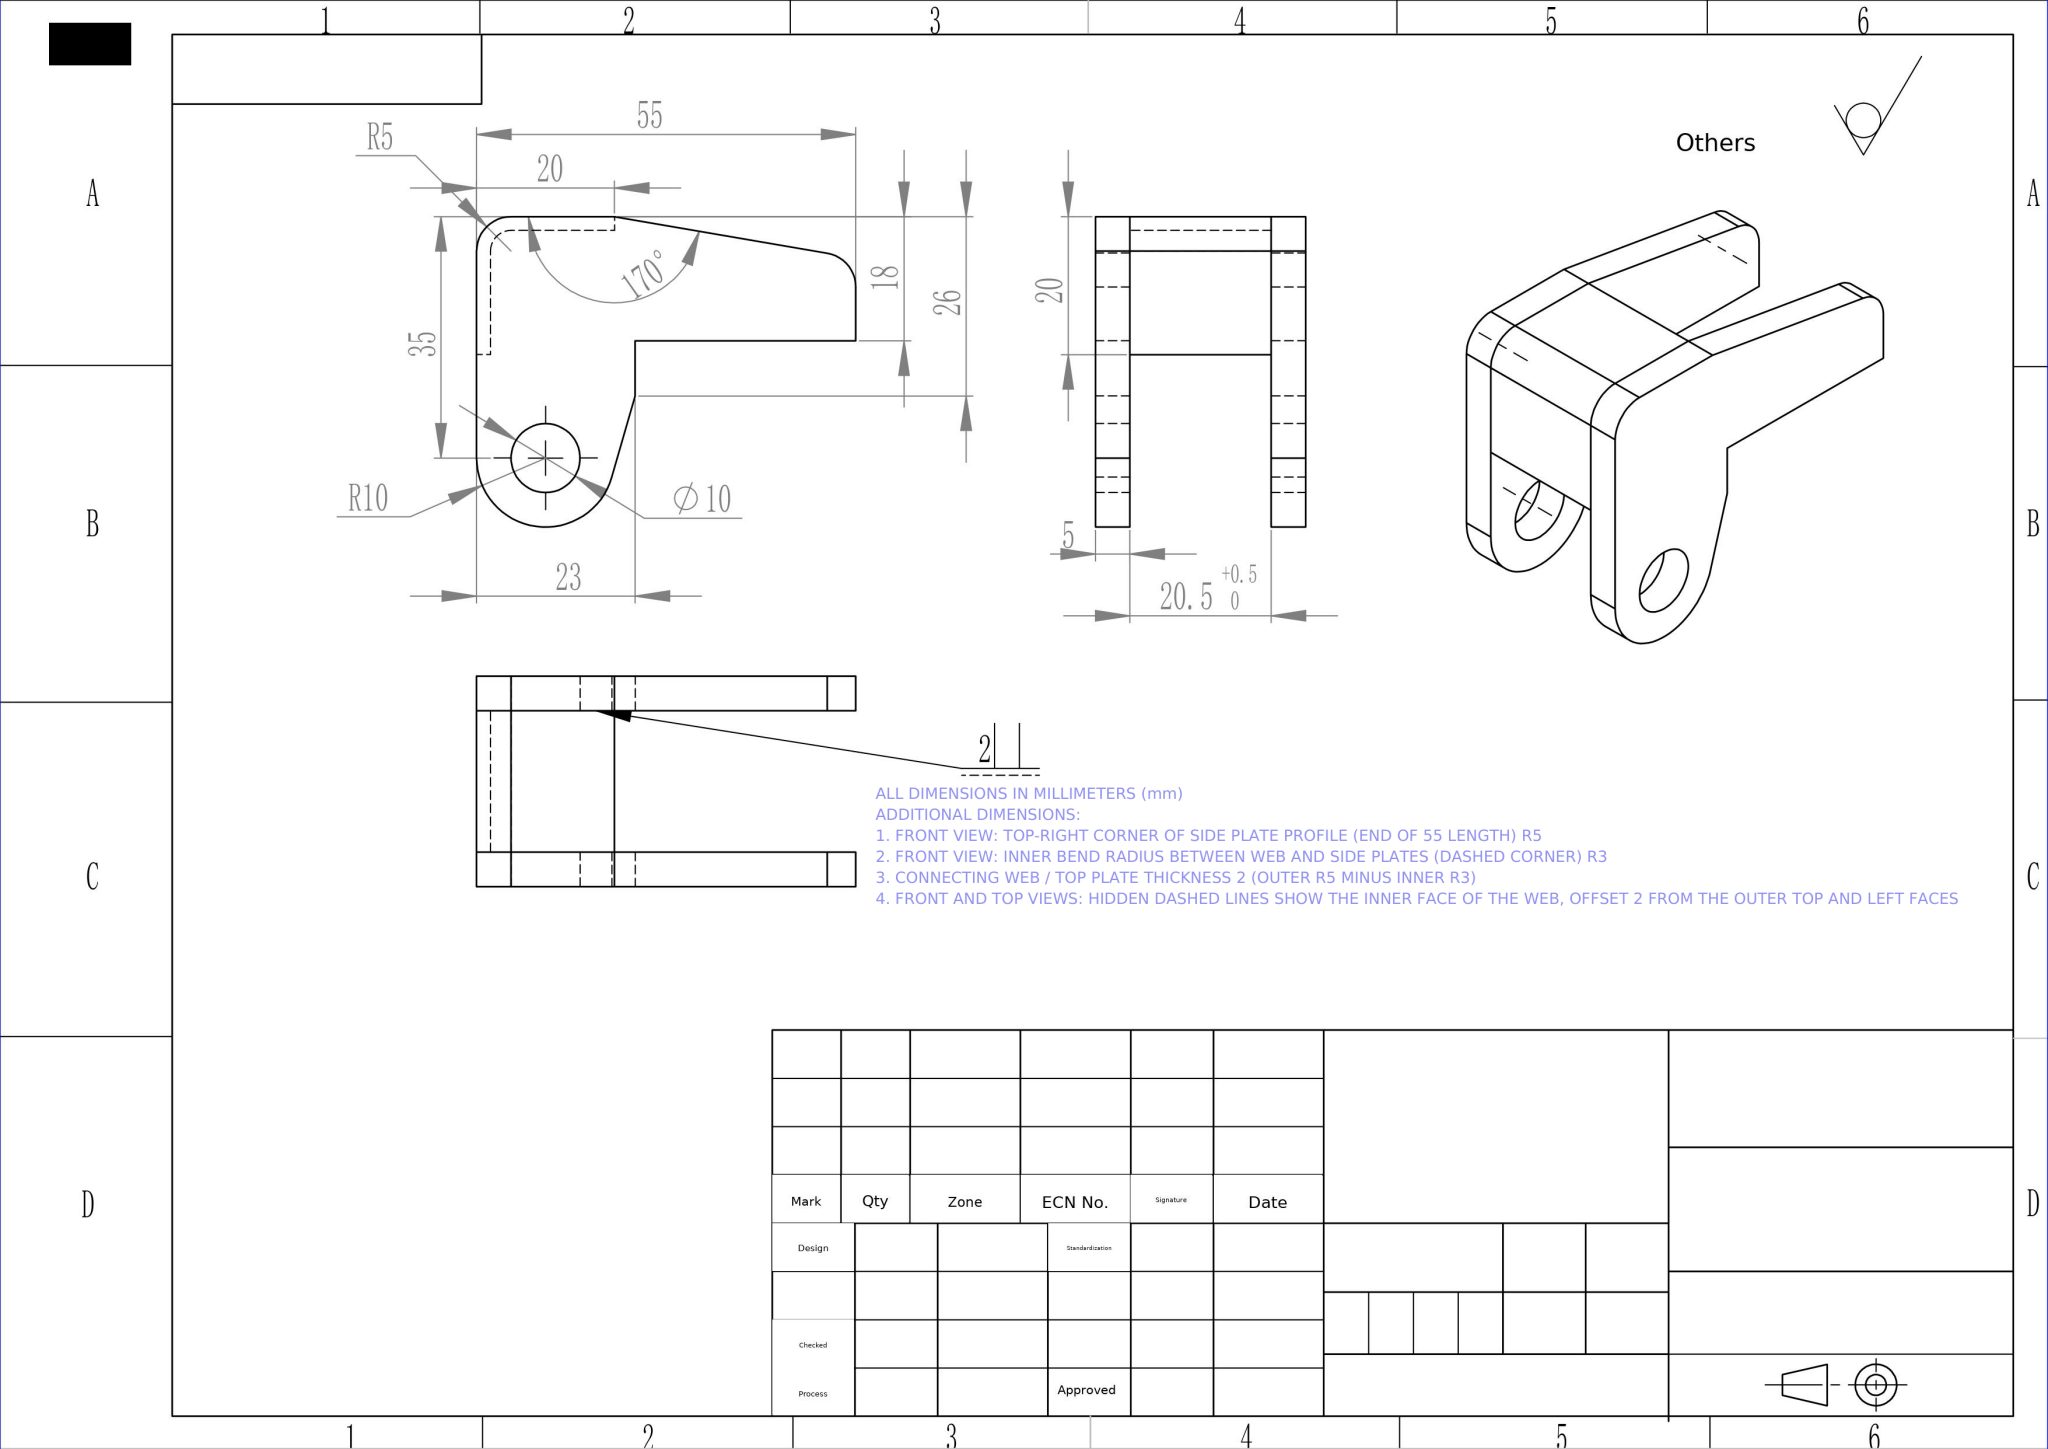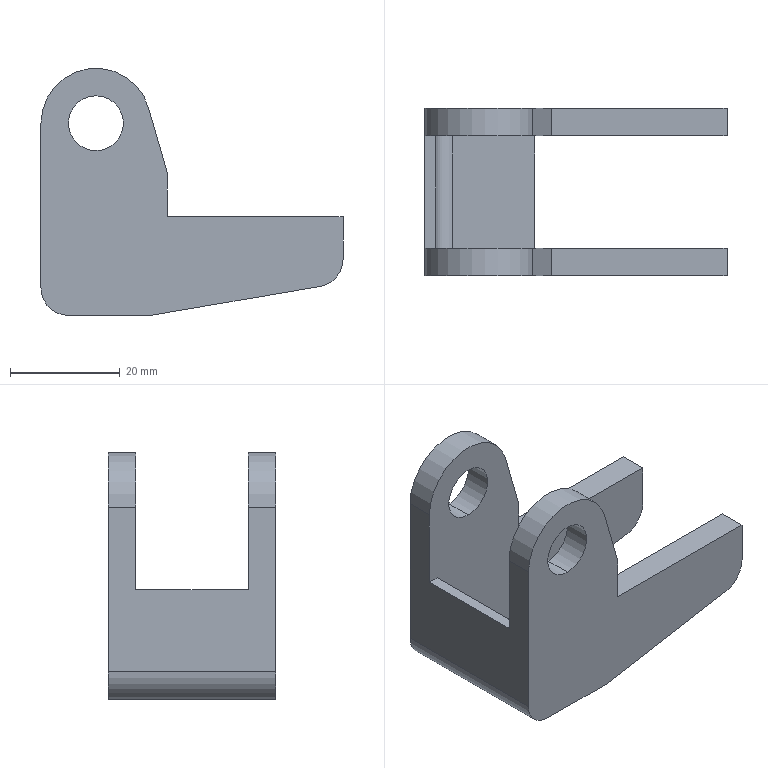Part | NX | mm | 1 solid | 30 faces | box 55 x 30.5 x 45 mm | volume 14831 mm3 | plane 20 | cylinder 10 | commonest cylinder face diameters 10 x7 20 x2 6 x1
STEP:
#1=COLOUR_RGB('',0.7922,0.8196,0.9333);
#2=FILL_AREA_STYLE_COLOUR('',#1);
#3=FILL_AREA_STYLE('',(#2));
#4=SURFACE_STYLE_FILL_AREA(#3);
#5=SURFACE_SIDE_STYLE('',(#4));
#6=SURFACE_STYLE_USAGE(.BOTH.,#5);
#7=PRESENTATION_STYLE_ASSIGNMENT((#6));
#8=CARTESIAN_POINT('',(5.,30.5,-35.));
#9=VERTEX_POINT('',#8);
#10=CARTESIAN_POINT('',(5.,0.,-35.));
#11=VERTEX_POINT('',#10);
#12=CARTESIAN_POINT('',(5.,25.5,-35.));
#13=DIRECTION('',(0.,-1.,0.));
#14=VECTOR('',#13,1000.);
#15=LINE('',#12,#14);
#16=EDGE_CURVE('',#9,#11,#15,.T.);
#17=ORIENTED_EDGE('',*,*,#16,.T.);
#18=CARTESIAN_POINT('',(-0.,0.,-30.));
#19=VERTEX_POINT('',#18);
#20=CARTESIAN_POINT('',(5.,0.,-30.));
#21=DIRECTION('',(0.,1.,0.));
#22=DIRECTION('',(0.,0.,1.));
#23=AXIS2_PLACEMENT_3D('',#20,#21,#22);
#24=CIRCLE('',#23,5.);
#25=EDGE_CURVE('',#11,#19,#24,.T.);
#26=ORIENTED_EDGE('',*,*,#25,.T.);
#27=CARTESIAN_POINT('',(-0.,30.5,-30.));
#28=VERTEX_POINT('',#27);
#29=CARTESIAN_POINT('',(-0.,25.5,-30.));
#30=DIRECTION('',(0.,-1.,0.));
#31=VECTOR('',#30,1000.);
#32=LINE('',#29,#31);
#33=EDGE_CURVE('',#28,#19,#32,.T.);
#34=ORIENTED_EDGE('',*,*,#33,.F.);
#35=CARTESIAN_POINT('',(5.,30.5,-30.));
#36=DIRECTION('',(0.,1.,0.));
#37=DIRECTION('',(0.,0.,1.));
#38=AXIS2_PLACEMENT_3D('',#35,#36,#37);
#39=CIRCLE('',#38,5.);
#40=EDGE_CURVE('',#9,#28,#39,.T.);
#41=ORIENTED_EDGE('',*,*,#40,.F.);
#42=EDGE_LOOP('',(#17,#26,#34,#41));
#43=FACE_OUTER_BOUND('',#42,.T.);
#44=CARTESIAN_POINT('',(5.,25.5,-30.));
#45=DIRECTION('',(0.,-1.,0.));
#46=DIRECTION('',(0.,0.,-1.));
#47=AXIS2_PLACEMENT_3D('',#44,#45,#46);
#48=CYLINDRICAL_SURFACE('',#47,5.);
#49=ADVANCED_FACE('',(#43),#48,.T.);
#50=CARTESIAN_POINT('',(20.,25.5,-35.));
#51=VERTEX_POINT('',#50);
#52=CARTESIAN_POINT('',(20.,5.,-35.));
#53=VERTEX_POINT('',#52);
#54=CARTESIAN_POINT('',(20.,25.5,-35.));
#55=DIRECTION('',(0.,-1.,0.));
#56=VECTOR('',#55,1000.);
#57=LINE('',#54,#56);
#58=EDGE_CURVE('',#51,#53,#57,.T.);
#59=ORIENTED_EDGE('',*,*,#58,.T.);
#60=CARTESIAN_POINT('',(20.,0.,-35.));
#61=VERTEX_POINT('',#60);
#62=CARTESIAN_POINT('',(20.,5.,-35.));
#63=DIRECTION('',(0.,-1.,0.));
#64=VECTOR('',#63,1000.);
#65=LINE('',#62,#64);
#66=EDGE_CURVE('',#53,#61,#65,.T.);
#67=ORIENTED_EDGE('',*,*,#66,.T.);
#68=CARTESIAN_POINT('',(20.,0.,-35.));
#69=DIRECTION('',(-1.,0.,0.));
#70=VECTOR('',#69,1000.);
#71=LINE('',#68,#70);
#72=EDGE_CURVE('',#61,#11,#71,.T.);
#73=ORIENTED_EDGE('',*,*,#72,.T.);
#74=ORIENTED_EDGE('',*,*,#16,.F.);
#75=CARTESIAN_POINT('',(20.,30.5,-35.));
#76=VERTEX_POINT('',#75);
#77=CARTESIAN_POINT('',(20.,30.5,-35.));
#78=DIRECTION('',(-1.,0.,0.));
#79=VECTOR('',#78,1000.);
#80=LINE('',#77,#79);
#81=EDGE_CURVE('',#76,#9,#80,.T.);
#82=ORIENTED_EDGE('',*,*,#81,.F.);
#83=CARTESIAN_POINT('',(20.,25.5,-35.));
#84=DIRECTION('',(0.,1.,0.));
#85=VECTOR('',#84,1000.);
#86=LINE('',#83,#85);
#87=EDGE_CURVE('',#51,#76,#86,.T.);
#88=ORIENTED_EDGE('',*,*,#87,.F.);
#89=EDGE_LOOP('',(#59,#67,#73,#74,#82,#88));
#90=FACE_OUTER_BOUND('',#89,.T.);
#91=CARTESIAN_POINT('',(5.,25.5,-35.));
#92=DIRECTION('',(0.,0.,1.));
#93=DIRECTION('',(1.,0.,0.));
#94=AXIS2_PLACEMENT_3D('',#91,#92,#93);
#95=PLANE('',#94);
#96=ADVANCED_FACE('',(#90),#95,.F.);
#97=CARTESIAN_POINT('',(20.,5.,-33.));
#98=VERTEX_POINT('',#97);
#99=CARTESIAN_POINT('',(20.,5.,-35.));
#100=DIRECTION('',(0.,0.,1.));
#101=VECTOR('',#100,1000.);
#102=LINE('',#99,#101);
#103=EDGE_CURVE('',#53,#98,#102,.T.);
#104=ORIENTED_EDGE('',*,*,#103,.F.);
#105=ORIENTED_EDGE('',*,*,#58,.F.);
#106=CARTESIAN_POINT('',(20.,25.5,-33.));
#107=VERTEX_POINT('',#106);
#108=CARTESIAN_POINT('',(20.,25.5,-35.));
#109=DIRECTION('',(0.,0.,1.));
#110=VECTOR('',#109,1000.);
#111=LINE('',#108,#110);
#112=EDGE_CURVE('',#51,#107,#111,.T.);
#113=ORIENTED_EDGE('',*,*,#112,.T.);
#114=CARTESIAN_POINT('',(20.,25.5,-33.));
#115=DIRECTION('',(0.,-1.,0.));
#116=VECTOR('',#115,1000.);
#117=LINE('',#114,#116);
#118=EDGE_CURVE('',#107,#98,#117,.T.);
#119=ORIENTED_EDGE('',*,*,#118,.T.);
#120=EDGE_LOOP('',(#104,#105,#113,#119));
#121=FACE_OUTER_BOUND('',#120,.T.);
#122=CARTESIAN_POINT('',(20.,25.5,-35.));
#123=DIRECTION('',(1.,0.,0.));
#124=DIRECTION('',(0.,1.,0.));
#125=AXIS2_PLACEMENT_3D('',#122,#123,#124);
#126=PLANE('',#125);
#127=ADVANCED_FACE('',(#121),#126,.T.);
#128=CARTESIAN_POINT('',(5.,5.,-33.));
#129=VERTEX_POINT('',#128);
#130=CARTESIAN_POINT('',(5.,5.,-33.));
#131=DIRECTION('',(-1.,0.,0.));
#132=VECTOR('',#131,1000.);
#133=LINE('',#130,#132);
#134=EDGE_CURVE('',#98,#129,#133,.T.);
#135=ORIENTED_EDGE('',*,*,#134,.F.);
#136=ORIENTED_EDGE('',*,*,#118,.F.);
#137=CARTESIAN_POINT('',(5.,25.5,-33.));
#138=VERTEX_POINT('',#137);
#139=CARTESIAN_POINT('',(5.,25.5,-33.));
#140=DIRECTION('',(-1.,0.,0.));
#141=VECTOR('',#140,1000.);
#142=LINE('',#139,#141);
#143=EDGE_CURVE('',#107,#138,#142,.T.);
#144=ORIENTED_EDGE('',*,*,#143,.T.);
#145=CARTESIAN_POINT('',(5.,25.5,-33.));
#146=DIRECTION('',(0.,-1.,0.));
#147=VECTOR('',#146,1000.);
#148=LINE('',#145,#147);
#149=EDGE_CURVE('',#138,#129,#148,.T.);
#150=ORIENTED_EDGE('',*,*,#149,.T.);
#151=EDGE_LOOP('',(#135,#136,#144,#150));
#152=FACE_OUTER_BOUND('',#151,.T.);
#153=CARTESIAN_POINT('',(5.,25.5,-33.));
#154=DIRECTION('',(0.,0.,1.));
#155=DIRECTION('',(1.,0.,0.));
#156=AXIS2_PLACEMENT_3D('',#153,#154,#155);
#157=PLANE('',#156);
#158=ADVANCED_FACE('',(#152),#157,.T.);
#159=CARTESIAN_POINT('',(2.,5.,-30.));
#160=VERTEX_POINT('',#159);
#161=CARTESIAN_POINT('',(5.,5.,-30.));
#162=DIRECTION('',(0.,1.,0.));
#163=DIRECTION('',(1.,0.,0.));
#164=AXIS2_PLACEMENT_3D('',#161,#162,#163);
#165=CIRCLE('',#164,3.);
#166=EDGE_CURVE('',#129,#160,#165,.T.);
#167=ORIENTED_EDGE('',*,*,#166,.F.);
#168=ORIENTED_EDGE('',*,*,#149,.F.);
#169=CARTESIAN_POINT('',(2.,25.5,-30.));
#170=VERTEX_POINT('',#169);
#171=CARTESIAN_POINT('',(5.,25.5,-30.));
#172=DIRECTION('',(0.,1.,0.));
#173=DIRECTION('',(1.,0.,0.));
#174=AXIS2_PLACEMENT_3D('',#171,#172,#173);
#175=CIRCLE('',#174,3.);
#176=EDGE_CURVE('',#138,#170,#175,.T.);
#177=ORIENTED_EDGE('',*,*,#176,.T.);
#178=CARTESIAN_POINT('',(2.,25.5,-30.));
#179=DIRECTION('',(0.,-1.,0.));
#180=VECTOR('',#179,1000.);
#181=LINE('',#178,#180);
#182=EDGE_CURVE('',#170,#160,#181,.T.);
#183=ORIENTED_EDGE('',*,*,#182,.T.);
#184=EDGE_LOOP('',(#167,#168,#177,#183));
#185=FACE_OUTER_BOUND('',#184,.T.);
#186=CARTESIAN_POINT('',(5.,25.5,-30.));
#187=DIRECTION('',(0.,-1.,0.));
#188=DIRECTION('',(0.,0.,-1.));
#189=AXIS2_PLACEMENT_3D('',#186,#187,#188);
#190=CYLINDRICAL_SURFACE('',#189,3.);
#191=ADVANCED_FACE('',(#185),#190,.F.);
#192=CARTESIAN_POINT('',(2.,5.,-15.));
#193=VERTEX_POINT('',#192);
#194=CARTESIAN_POINT('',(2.,5.,-30.));
#195=DIRECTION('',(0.,0.,1.));
#196=VECTOR('',#195,1000.);
#197=LINE('',#194,#196);
#198=EDGE_CURVE('',#160,#193,#197,.T.);
#199=ORIENTED_EDGE('',*,*,#198,.F.);
#200=ORIENTED_EDGE('',*,*,#182,.F.);
#201=CARTESIAN_POINT('',(2.,25.5,-15.));
#202=VERTEX_POINT('',#201);
#203=CARTESIAN_POINT('',(2.,25.5,-30.));
#204=DIRECTION('',(0.,0.,1.));
#205=VECTOR('',#204,1000.);
#206=LINE('',#203,#205);
#207=EDGE_CURVE('',#170,#202,#206,.T.);
#208=ORIENTED_EDGE('',*,*,#207,.T.);
#209=CARTESIAN_POINT('',(2.,25.5,-15.));
#210=DIRECTION('',(0.,-1.,0.));
#211=VECTOR('',#210,1000.);
#212=LINE('',#209,#211);
#213=EDGE_CURVE('',#202,#193,#212,.T.);
#214=ORIENTED_EDGE('',*,*,#213,.T.);
#215=EDGE_LOOP('',(#199,#200,#208,#214));
#216=FACE_OUTER_BOUND('',#215,.T.);
#217=CARTESIAN_POINT('',(2.,25.5,-30.));
#218=DIRECTION('',(1.,0.,-0.));
#219=DIRECTION('',(-0.,0.,-1.));
#220=AXIS2_PLACEMENT_3D('',#217,#218,#219);
#221=PLANE('',#220);
#222=ADVANCED_FACE('',(#216),#221,.T.);
#223=CARTESIAN_POINT('',(-0.,5.,-15.));
#224=VERTEX_POINT('',#223);
#225=CARTESIAN_POINT('',(2.,5.,-15.));
#226=DIRECTION('',(-1.,0.,0.));
#227=VECTOR('',#226,1000.);
#228=LINE('',#225,#227);
#229=EDGE_CURVE('',#193,#224,#228,.T.);
#230=ORIENTED_EDGE('',*,*,#229,.F.);
#231=ORIENTED_EDGE('',*,*,#213,.F.);
#232=CARTESIAN_POINT('',(-0.,25.5,-15.));
#233=VERTEX_POINT('',#232);
#234=CARTESIAN_POINT('',(2.,25.5,-15.));
#235=DIRECTION('',(-1.,0.,0.));
#236=VECTOR('',#235,1000.);
#237=LINE('',#234,#236);
#238=EDGE_CURVE('',#202,#233,#237,.T.);
#239=ORIENTED_EDGE('',*,*,#238,.T.);
#240=CARTESIAN_POINT('',(0.,25.5,-15.));
#241=DIRECTION('',(0.,-1.,0.));
#242=VECTOR('',#241,1000.);
#243=LINE('',#240,#242);
#244=EDGE_CURVE('',#233,#224,#243,.T.);
#245=ORIENTED_EDGE('',*,*,#244,.T.);
#246=EDGE_LOOP('',(#230,#231,#239,#245));
#247=FACE_OUTER_BOUND('',#246,.T.);
#248=CARTESIAN_POINT('',(2.,25.5,-15.));
#249=DIRECTION('',(0.,0.,1.));
#250=DIRECTION('',(1.,0.,0.));
#251=AXIS2_PLACEMENT_3D('',#248,#249,#250);
#252=PLANE('',#251);
#253=ADVANCED_FACE('',(#247),#252,.T.);
#254=ORIENTED_EDGE('',*,*,#33,.T.);
#255=CARTESIAN_POINT('',(0.,0.,0.));
#256=VERTEX_POINT('',#255);
#257=CARTESIAN_POINT('',(-0.,0.,-30.));
#258=DIRECTION('',(0.,0.,1.));
#259=VECTOR('',#258,1000.);
#260=LINE('',#257,#259);
#261=EDGE_CURVE('',#19,#256,#260,.T.);
#262=ORIENTED_EDGE('',*,*,#261,.T.);
#263=CARTESIAN_POINT('',(0.,5.,0.));
#264=VERTEX_POINT('',#263);
#265=CARTESIAN_POINT('',(0.,5.,0.));
#266=DIRECTION('',(0.,-1.,0.));
#267=VECTOR('',#266,1000.);
#268=LINE('',#265,#267);
#269=EDGE_CURVE('',#264,#256,#268,.T.);
#270=ORIENTED_EDGE('',*,*,#269,.F.);
#271=CARTESIAN_POINT('',(-0.,5.,-30.));
#272=DIRECTION('',(0.,0.,1.));
#273=VECTOR('',#272,1000.);
#274=LINE('',#271,#273);
#275=EDGE_CURVE('',#224,#264,#274,.T.);
#276=ORIENTED_EDGE('',*,*,#275,.F.);
#277=ORIENTED_EDGE('',*,*,#244,.F.);
#278=CARTESIAN_POINT('',(0.,25.5,0.));
#279=VERTEX_POINT('',#278);
#280=CARTESIAN_POINT('',(-0.,25.5,-30.));
#281=DIRECTION('',(0.,0.,1.));
#282=VECTOR('',#281,1000.);
#283=LINE('',#280,#282);
#284=EDGE_CURVE('',#233,#279,#283,.T.);
#285=ORIENTED_EDGE('',*,*,#284,.T.);
#286=CARTESIAN_POINT('',(0.,30.5,0.));
#287=VERTEX_POINT('',#286);
#288=CARTESIAN_POINT('',(0.,25.5,0.));
#289=DIRECTION('',(0.,1.,0.));
#290=VECTOR('',#289,1000.);
#291=LINE('',#288,#290);
#292=EDGE_CURVE('',#279,#287,#291,.T.);
#293=ORIENTED_EDGE('',*,*,#292,.T.);
#294=CARTESIAN_POINT('',(-0.,30.5,-30.));
#295=DIRECTION('',(0.,0.,1.));
#296=VECTOR('',#295,1000.);
#297=LINE('',#294,#296);
#298=EDGE_CURVE('',#28,#287,#297,.T.);
#299=ORIENTED_EDGE('',*,*,#298,.F.);
#300=EDGE_LOOP('',(#254,#262,#270,#276,#277,#285,#293,#299));
#301=FACE_OUTER_BOUND('',#300,.T.);
#302=CARTESIAN_POINT('',(-0.,25.5,-30.));
#303=DIRECTION('',(1.,0.,-0.));
#304=DIRECTION('',(-0.,0.,-1.));
#305=AXIS2_PLACEMENT_3D('',#302,#303,#304);
#306=PLANE('',#305);
#307=ADVANCED_FACE('',(#301),#306,.F.);
#308=CARTESIAN_POINT('',(10.,25.5,-5.));
#309=VERTEX_POINT('',#308);
#310=CARTESIAN_POINT('',(10.,25.5,5.));
#311=VERTEX_POINT('',#310);
#312=CARTESIAN_POINT('',(10.,25.5,0.));
#313=DIRECTION('',(0.,1.,0.));
#314=DIRECTION('',(0.,0.,1.));
#315=AXIS2_PLACEMENT_3D('',#312,#313,#314);
#316=CIRCLE('',#315,5.);
#317=EDGE_CURVE('',#309,#311,#316,.T.);
#318=ORIENTED_EDGE('',*,*,#317,.T.);
#319=CARTESIAN_POINT('',(10.,25.5,0.));
#320=DIRECTION('',(0.,1.,0.));
#321=DIRECTION('',(0.,0.,1.));
#322=AXIS2_PLACEMENT_3D('',#319,#320,#321);
#323=CIRCLE('',#322,5.);
#324=EDGE_CURVE('',#311,#309,#323,.T.);
#325=ORIENTED_EDGE('',*,*,#324,.T.);
#326=EDGE_LOOP('',(#318,#325));
#327=FACE_BOUND('',#326,.T.);
#328=ORIENTED_EDGE('',*,*,#238,.F.);
#329=ORIENTED_EDGE('',*,*,#207,.F.);
#330=ORIENTED_EDGE('',*,*,#176,.F.);
#331=ORIENTED_EDGE('',*,*,#143,.F.);
#332=ORIENTED_EDGE('',*,*,#112,.F.);
#333=CARTESIAN_POINT('',(50.845,25.5,-29.712));
#334=VERTEX_POINT('',#333);
#335=CARTESIAN_POINT('',(50.845,25.5,-29.712));
#336=DIRECTION('',(-0.9856,0.,-0.169));
#337=VECTOR('',#336,1000.);
#338=LINE('',#335,#337);
#339=EDGE_CURVE('',#334,#51,#338,.T.);
#340=ORIENTED_EDGE('',*,*,#339,.F.);
#341=CARTESIAN_POINT('',(55.,25.5,-24.784));
#342=VERTEX_POINT('',#341);
#343=CARTESIAN_POINT('',(50.,25.5,-24.784));
#344=DIRECTION('',(0.,1.,0.));
#345=DIRECTION('',(0.,0.,1.));
#346=AXIS2_PLACEMENT_3D('',#343,#344,#345);
#347=CIRCLE('',#346,5.);
#348=EDGE_CURVE('',#342,#334,#347,.T.);
#349=ORIENTED_EDGE('',*,*,#348,.F.);
#350=CARTESIAN_POINT('',(55.,25.5,-17.));
#351=VERTEX_POINT('',#350);
#352=CARTESIAN_POINT('',(55.,25.5,-17.));
#353=DIRECTION('',(-0.,0.,-1.));
#354=VECTOR('',#353,1000.);
#355=LINE('',#352,#354);
#356=EDGE_CURVE('',#351,#342,#355,.T.);
#357=ORIENTED_EDGE('',*,*,#356,.F.);
#358=CARTESIAN_POINT('',(23.,25.5,-17.));
#359=VERTEX_POINT('',#358);
#360=CARTESIAN_POINT('',(23.,25.5,-17.));
#361=DIRECTION('',(1.,0.,0.));
#362=VECTOR('',#361,1000.);
#363=LINE('',#360,#362);
#364=EDGE_CURVE('',#359,#351,#363,.T.);
#365=ORIENTED_EDGE('',*,*,#364,.F.);
#366=CARTESIAN_POINT('',(23.,25.5,-9.));
#367=VERTEX_POINT('',#366);
#368=CARTESIAN_POINT('',(23.,25.5,-9.));
#369=DIRECTION('',(0.,0.,-1.));
#370=VECTOR('',#369,1000.);
#371=LINE('',#368,#370);
#372=EDGE_CURVE('',#367,#359,#371,.T.);
#373=ORIENTED_EDGE('',*,*,#372,.F.);
#374=CARTESIAN_POINT('',(19.609,25.5,2.769));
#375=VERTEX_POINT('',#374);
#376=CARTESIAN_POINT('',(23.,25.5,-9.));
#377=DIRECTION('',(0.2769,0.,-0.9609));
#378=VECTOR('',#377,1000.);
#379=LINE('',#376,#378);
#380=EDGE_CURVE('',#375,#367,#379,.T.);
#381=ORIENTED_EDGE('',*,*,#380,.F.);
#382=CARTESIAN_POINT('',(10.,25.5,0.));
#383=DIRECTION('',(0.,1.,0.));
#384=DIRECTION('',(0.,0.,1.));
#385=AXIS2_PLACEMENT_3D('',#382,#383,#384);
#386=CIRCLE('',#385,10.);
#387=EDGE_CURVE('',#279,#375,#386,.T.);
#388=ORIENTED_EDGE('',*,*,#387,.F.);
#389=ORIENTED_EDGE('',*,*,#284,.F.);
#390=EDGE_LOOP('',(#328,#329,#330,#331,#332,#340,#349,#357,#365,#373,#381,#388,#389));
#391=FACE_OUTER_BOUND('',#390,.T.);
#392=CARTESIAN_POINT('',(10.,25.5,0.));
#393=DIRECTION('',(0.,-1.,0.));
#394=DIRECTION('',(0.,0.,-1.));
#395=AXIS2_PLACEMENT_3D('',#392,#393,#394);
#396=PLANE('',#395);
#397=ADVANCED_FACE('',(#327,#391),#396,.T.);
#398=CARTESIAN_POINT('',(10.,30.5,5.));
#399=VERTEX_POINT('',#398);
#400=CARTESIAN_POINT('',(10.,25.5,5.));
#401=DIRECTION('',(0.,1.,0.));
#402=VECTOR('',#401,1000.);
#403=LINE('',#400,#402);
#404=EDGE_CURVE('',#311,#399,#403,.T.);
#405=ORIENTED_EDGE('',*,*,#404,.F.);
#406=ORIENTED_EDGE('',*,*,#317,.F.);
#407=CARTESIAN_POINT('',(10.,30.5,-5.));
#408=VERTEX_POINT('',#407);
#409=CARTESIAN_POINT('',(10.,25.5,-5.));
#410=DIRECTION('',(0.,1.,0.));
#411=VECTOR('',#410,1000.);
#412=LINE('',#409,#411);
#413=EDGE_CURVE('',#309,#408,#412,.T.);
#414=ORIENTED_EDGE('',*,*,#413,.T.);
#415=CARTESIAN_POINT('',(10.,30.5,0.));
#416=DIRECTION('',(0.,1.,0.));
#417=DIRECTION('',(0.,0.,1.));
#418=AXIS2_PLACEMENT_3D('',#415,#416,#417);
#419=CIRCLE('',#418,5.);
#420=EDGE_CURVE('',#408,#399,#419,.T.);
#421=ORIENTED_EDGE('',*,*,#420,.T.);
#422=EDGE_LOOP('',(#405,#406,#414,#421));
#423=FACE_OUTER_BOUND('',#422,.T.);
#424=CARTESIAN_POINT('',(10.,25.5,0.));
#425=DIRECTION('',(0.,1.,0.));
#426=DIRECTION('',(0.,0.,-1.));
#427=AXIS2_PLACEMENT_3D('',#424,#425,#426);
#428=CYLINDRICAL_SURFACE('',#427,5.);
#429=ADVANCED_FACE('',(#423),#428,.F.);
#430=CARTESIAN_POINT('',(50.845,30.5,-29.712));
#431=VERTEX_POINT('',#430);
#432=CARTESIAN_POINT('',(50.845,30.5,-29.712));
#433=DIRECTION('',(-0.9856,0.,-0.169));
#434=VECTOR('',#433,1000.);
#435=LINE('',#432,#434);
#436=EDGE_CURVE('',#431,#76,#435,.T.);
#437=ORIENTED_EDGE('',*,*,#436,.F.);
#438=CARTESIAN_POINT('',(50.845,25.5,-29.712));
#439=DIRECTION('',(0.,1.,0.));
#440=VECTOR('',#439,1000.);
#441=LINE('',#438,#440);
#442=EDGE_CURVE('',#334,#431,#441,.T.);
#443=ORIENTED_EDGE('',*,*,#442,.F.);
#444=ORIENTED_EDGE('',*,*,#339,.T.);
#445=ORIENTED_EDGE('',*,*,#87,.T.);
#446=EDGE_LOOP('',(#437,#443,#444,#445));
#447=FACE_OUTER_BOUND('',#446,.T.);
#448=CARTESIAN_POINT('',(50.845,25.5,-29.712));
#449=DIRECTION('',(-0.169,0.,0.9856));
#450=DIRECTION('',(0.,1.,0.));
#451=AXIS2_PLACEMENT_3D('',#448,#449,#450);
#452=PLANE('',#451);
#453=ADVANCED_FACE('',(#447),#452,.F.);
#454=CARTESIAN_POINT('',(55.,30.5,-24.784));
#455=VERTEX_POINT('',#454);
#456=CARTESIAN_POINT('',(50.,30.5,-24.784));
#457=DIRECTION('',(0.,1.,0.));
#458=DIRECTION('',(0.,0.,1.));
#459=AXIS2_PLACEMENT_3D('',#456,#457,#458);
#460=CIRCLE('',#459,5.);
#461=EDGE_CURVE('',#455,#431,#460,.T.);
#462=ORIENTED_EDGE('',*,*,#461,.F.);
#463=CARTESIAN_POINT('',(55.,25.5,-24.784));
#464=DIRECTION('',(0.,1.,0.));
#465=VECTOR('',#464,1000.);
#466=LINE('',#463,#465);
#467=EDGE_CURVE('',#342,#455,#466,.T.);
#468=ORIENTED_EDGE('',*,*,#467,.F.);
#469=ORIENTED_EDGE('',*,*,#348,.T.);
#470=ORIENTED_EDGE('',*,*,#442,.T.);
#471=EDGE_LOOP('',(#462,#468,#469,#470));
#472=FACE_OUTER_BOUND('',#471,.T.);
#473=CARTESIAN_POINT('',(50.,25.5,-24.784));
#474=DIRECTION('',(0.,1.,0.));
#475=DIRECTION('',(0.,0.,-1.));
#476=AXIS2_PLACEMENT_3D('',#473,#474,#475);
#477=CYLINDRICAL_SURFACE('',#476,5.);
#478=ADVANCED_FACE('',(#472),#477,.T.);
#479=CARTESIAN_POINT('',(55.,30.5,-17.));
#480=VERTEX_POINT('',#479);
#481=CARTESIAN_POINT('',(55.,30.5,-17.));
#482=DIRECTION('',(-0.,0.,-1.));
#483=VECTOR('',#482,1000.);
#484=LINE('',#481,#483);
#485=EDGE_CURVE('',#480,#455,#484,.T.);
#486=ORIENTED_EDGE('',*,*,#485,.F.);
#487=CARTESIAN_POINT('',(55.,25.5,-17.));
#488=DIRECTION('',(0.,1.,0.));
#489=VECTOR('',#488,1000.);
#490=LINE('',#487,#489);
#491=EDGE_CURVE('',#351,#480,#490,.T.);
#492=ORIENTED_EDGE('',*,*,#491,.F.);
#493=ORIENTED_EDGE('',*,*,#356,.T.);
#494=ORIENTED_EDGE('',*,*,#467,.T.);
#495=EDGE_LOOP('',(#486,#492,#493,#494));
#496=FACE_OUTER_BOUND('',#495,.T.);
#497=CARTESIAN_POINT('',(55.,25.5,-17.));
#498=DIRECTION('',(-1.,0.,0.));
#499=DIRECTION('',(0.,1.,0.));
#500=AXIS2_PLACEMENT_3D('',#497,#498,#499);
#501=PLANE('',#500);
#502=ADVANCED_FACE('',(#496),#501,.F.);
#503=CARTESIAN_POINT('',(23.,30.5,-17.));
#504=VERTEX_POINT('',#503);
#505=CARTESIAN_POINT('',(23.,30.5,-17.));
#506=DIRECTION('',(1.,0.,0.));
#507=VECTOR('',#506,1000.);
#508=LINE('',#505,#507);
#509=EDGE_CURVE('',#504,#480,#508,.T.);
#510=ORIENTED_EDGE('',*,*,#509,.F.);
#511=CARTESIAN_POINT('',(23.,25.5,-17.));
#512=DIRECTION('',(0.,1.,0.));
#513=VECTOR('',#512,1000.);
#514=LINE('',#511,#513);
#515=EDGE_CURVE('',#359,#504,#514,.T.);
#516=ORIENTED_EDGE('',*,*,#515,.F.);
#517=ORIENTED_EDGE('',*,*,#364,.T.);
#518=ORIENTED_EDGE('',*,*,#491,.T.);
#519=EDGE_LOOP('',(#510,#516,#517,#518));
#520=FACE_OUTER_BOUND('',#519,.T.);
#521=CARTESIAN_POINT('',(23.,25.5,-17.));
#522=DIRECTION('',(0.,0.,-1.));
#523=DIRECTION('',(0.,-1.,0.));
#524=AXIS2_PLACEMENT_3D('',#521,#522,#523);
#525=PLANE('',#524);
#526=ADVANCED_FACE('',(#520),#525,.F.);
#527=CARTESIAN_POINT('',(23.,30.5,-9.));
#528=VERTEX_POINT('',#527);
#529=CARTESIAN_POINT('',(23.,30.5,-9.));
#530=DIRECTION('',(0.,0.,-1.));
#531=VECTOR('',#530,1000.);
#532=LINE('',#529,#531);
#533=EDGE_CURVE('',#528,#504,#532,.T.);
#534=ORIENTED_EDGE('',*,*,#533,.F.);
#535=CARTESIAN_POINT('',(23.,25.5,-9.));
#536=DIRECTION('',(0.,1.,0.));
#537=VECTOR('',#536,1000.);
#538=LINE('',#535,#537);
#539=EDGE_CURVE('',#367,#528,#538,.T.);
#540=ORIENTED_EDGE('',*,*,#539,.F.);
#541=ORIENTED_EDGE('',*,*,#372,.T.);
#542=ORIENTED_EDGE('',*,*,#515,.T.);
#543=EDGE_LOOP('',(#534,#540,#541,#542));
#544=FACE_OUTER_BOUND('',#543,.T.);
#545=CARTESIAN_POINT('',(23.,25.5,-9.));
#546=DIRECTION('',(-1.,0.,0.));
#547=DIRECTION('',(0.,0.,1.));
#548=AXIS2_PLACEMENT_3D('',#545,#546,#547);
#549=PLANE('',#548);
#550=ADVANCED_FACE('',(#544),#549,.F.);
#551=CARTESIAN_POINT('',(19.609,30.5,2.769));
#552=VERTEX_POINT('',#551);
#553=CARTESIAN_POINT('',(23.,30.5,-9.));
#554=DIRECTION('',(0.2769,0.,-0.9609));
#555=VECTOR('',#554,1000.);
#556=LINE('',#553,#555);
#557=EDGE_CURVE('',#552,#528,#556,.T.);
#558=ORIENTED_EDGE('',*,*,#557,.F.);
#559=CARTESIAN_POINT('',(19.609,25.5,2.769));
#560=DIRECTION('',(0.,1.,0.));
#561=VECTOR('',#560,1000.);
#562=LINE('',#559,#561);
#563=EDGE_CURVE('',#375,#552,#562,.T.);
#564=ORIENTED_EDGE('',*,*,#563,.F.);
#565=ORIENTED_EDGE('',*,*,#380,.T.);
#566=ORIENTED_EDGE('',*,*,#539,.T.);
#567=EDGE_LOOP('',(#558,#564,#565,#566));
#568=FACE_OUTER_BOUND('',#567,.T.);
#569=CARTESIAN_POINT('',(23.,25.5,-9.));
#570=DIRECTION('',(-0.9609,0.,-0.2769));
#571=DIRECTION('',(-0.2769,0.,0.9609));
#572=AXIS2_PLACEMENT_3D('',#569,#570,#571);
#573=PLANE('',#572);
#574=ADVANCED_FACE('',(#568),#573,.F.);
#575=CARTESIAN_POINT('',(10.,30.5,0.));
#576=DIRECTION('',(0.,1.,0.));
#577=DIRECTION('',(0.,0.,1.));
#578=AXIS2_PLACEMENT_3D('',#575,#576,#577);
#579=CIRCLE('',#578,10.);
#580=EDGE_CURVE('',#287,#552,#579,.T.);
#581=ORIENTED_EDGE('',*,*,#580,.F.);
#582=ORIENTED_EDGE('',*,*,#292,.F.);
#583=ORIENTED_EDGE('',*,*,#387,.T.);
#584=ORIENTED_EDGE('',*,*,#563,.T.);
#585=EDGE_LOOP('',(#581,#582,#583,#584));
#586=FACE_OUTER_BOUND('',#585,.T.);
#587=CARTESIAN_POINT('',(10.,25.5,0.));
#588=DIRECTION('',(0.,1.,0.));
#589=DIRECTION('',(0.,0.,-1.));
#590=AXIS2_PLACEMENT_3D('',#587,#588,#589);
#591=CYLINDRICAL_SURFACE('',#590,10.);
#592=ADVANCED_FACE('',(#586),#591,.T.);
#593=ORIENTED_EDGE('',*,*,#420,.F.);
#594=CARTESIAN_POINT('',(10.,30.5,0.));
#595=DIRECTION('',(0.,1.,0.));
#596=DIRECTION('',(0.,0.,1.));
#597=AXIS2_PLACEMENT_3D('',#594,#595,#596);
#598=CIRCLE('',#597,5.);
#599=EDGE_CURVE('',#399,#408,#598,.T.);
#600=ORIENTED_EDGE('',*,*,#599,.F.);
#601=EDGE_LOOP('',(#593,#600));
#602=FACE_BOUND('',#601,.T.);
#603=ORIENTED_EDGE('',*,*,#580,.T.);
#604=ORIENTED_EDGE('',*,*,#557,.T.);
#605=ORIENTED_EDGE('',*,*,#533,.T.);
#606=ORIENTED_EDGE('',*,*,#509,.T.);
#607=ORIENTED_EDGE('',*,*,#485,.T.);
#608=ORIENTED_EDGE('',*,*,#461,.T.);
#609=ORIENTED_EDGE('',*,*,#436,.T.);
#610=ORIENTED_EDGE('',*,*,#81,.T.);
#611=ORIENTED_EDGE('',*,*,#40,.T.);
#612=ORIENTED_EDGE('',*,*,#298,.T.);
#613=EDGE_LOOP('',(#603,#604,#605,#606,#607,#608,#609,#610,#611,#612));
#614=FACE_OUTER_BOUND('',#613,.T.);
#615=CARTESIAN_POINT('',(10.,30.5,0.));
#616=DIRECTION('',(0.,-1.,0.));
#617=DIRECTION('',(0.,0.,-1.));
#618=AXIS2_PLACEMENT_3D('',#615,#616,#617);
#619=PLANE('',#618);
#620=ADVANCED_FACE('',(#602,#614),#619,.F.);
#621=ORIENTED_EDGE('',*,*,#324,.F.);
#622=ORIENTED_EDGE('',*,*,#404,.T.);
#623=ORIENTED_EDGE('',*,*,#599,.T.);
#624=ORIENTED_EDGE('',*,*,#413,.F.);
#625=EDGE_LOOP('',(#621,#622,#623,#624));
#626=FACE_OUTER_BOUND('',#625,.T.);
#627=CARTESIAN_POINT('',(10.,25.5,0.));
#628=DIRECTION('',(0.,1.,0.));
#629=DIRECTION('',(0.,0.,-1.));
#630=AXIS2_PLACEMENT_3D('',#627,#628,#629);
#631=CYLINDRICAL_SURFACE('',#630,5.);
#632=ADVANCED_FACE('',(#626),#631,.F.);
#633=CARTESIAN_POINT('',(10.,5.,5.));
#634=VERTEX_POINT('',#633);
#635=CARTESIAN_POINT('',(10.,0.,5.));
#636=VERTEX_POINT('',#635);
#637=CARTESIAN_POINT('',(10.,5.,5.));
#638=DIRECTION('',(0.,-1.,0.));
#639=VECTOR('',#638,1000.);
#640=LINE('',#637,#639);
#641=EDGE_CURVE('',#634,#636,#640,.T.);
#642=ORIENTED_EDGE('',*,*,#641,.F.);
#643=CARTESIAN_POINT('',(10.,5.,-5.));
#644=VERTEX_POINT('',#643);
#645=CARTESIAN_POINT('',(10.,5.,0.));
#646=DIRECTION('',(0.,1.,0.));
#647=DIRECTION('',(0.,0.,1.));
#648=AXIS2_PLACEMENT_3D('',#645,#646,#647);
#649=CIRCLE('',#648,5.);
#650=EDGE_CURVE('',#634,#644,#649,.T.);
#651=ORIENTED_EDGE('',*,*,#650,.T.);
#652=CARTESIAN_POINT('',(10.,0.,-5.));
#653=VERTEX_POINT('',#652);
#654=CARTESIAN_POINT('',(10.,5.,-5.));
#655=DIRECTION('',(0.,-1.,0.));
#656=VECTOR('',#655,1000.);
#657=LINE('',#654,#656);
#658=EDGE_CURVE('',#644,#653,#657,.T.);
#659=ORIENTED_EDGE('',*,*,#658,.T.);
#660=CARTESIAN_POINT('',(10.,0.,0.));
#661=DIRECTION('',(0.,1.,0.));
#662=DIRECTION('',(0.,0.,1.));
#663=AXIS2_PLACEMENT_3D('',#660,#661,#662);
#664=CIRCLE('',#663,5.);
#665=EDGE_CURVE('',#636,#653,#664,.T.);
#666=ORIENTED_EDGE('',*,*,#665,.F.);
#667=EDGE_LOOP('',(#642,#651,#659,#666));
#668=FACE_OUTER_BOUND('',#667,.T.);
#669=CARTESIAN_POINT('',(10.,5.,0.));
#670=DIRECTION('',(0.,-1.,0.));
#671=DIRECTION('',(0.,0.,-1.));
#672=AXIS2_PLACEMENT_3D('',#669,#670,#671);
#673=CYLINDRICAL_SURFACE('',#672,5.);
#674=ADVANCED_FACE('',(#668),#673,.F.);
#675=CARTESIAN_POINT('',(50.845,0.,-29.712));
#676=VERTEX_POINT('',#675);
#677=CARTESIAN_POINT('',(50.845,0.,-29.712));
#678=DIRECTION('',(-0.9856,0.,-0.169));
#679=VECTOR('',#678,1000.);
#680=LINE('',#677,#679);
#681=EDGE_CURVE('',#676,#61,#680,.T.);
#682=ORIENTED_EDGE('',*,*,#681,.T.);
#683=ORIENTED_EDGE('',*,*,#66,.F.);
#684=CARTESIAN_POINT('',(50.845,5.,-29.712));
#685=VERTEX_POINT('',#684);
#686=CARTESIAN_POINT('',(50.845,5.,-29.712));
#687=DIRECTION('',(-0.9856,0.,-0.169));
#688=VECTOR('',#687,1000.);
#689=LINE('',#686,#688);
#690=EDGE_CURVE('',#685,#53,#689,.T.);
#691=ORIENTED_EDGE('',*,*,#690,.F.);
#692=CARTESIAN_POINT('',(50.845,5.,-29.712));
#693=DIRECTION('',(0.,-1.,0.));
#694=VECTOR('',#693,1000.);
#695=LINE('',#692,#694);
#696=EDGE_CURVE('',#685,#676,#695,.T.);
#697=ORIENTED_EDGE('',*,*,#696,.T.);
#698=EDGE_LOOP('',(#682,#683,#691,#697));
#699=FACE_OUTER_BOUND('',#698,.T.);
#700=CARTESIAN_POINT('',(50.845,5.,-29.712));
#701=DIRECTION('',(-0.169,0.,0.9856));
#702=DIRECTION('',(0.,1.,0.));
#703=AXIS2_PLACEMENT_3D('',#700,#701,#702);
#704=PLANE('',#703);
#705=ADVANCED_FACE('',(#699),#704,.F.);
#706=CARTESIAN_POINT('',(55.,0.,-24.784));
#707=VERTEX_POINT('',#706);
#708=CARTESIAN_POINT('',(50.,0.,-24.784));
#709=DIRECTION('',(0.,1.,0.));
#710=DIRECTION('',(0.,0.,1.));
#711=AXIS2_PLACEMENT_3D('',#708,#709,#710);
#712=CIRCLE('',#711,5.);
#713=EDGE_CURVE('',#707,#676,#712,.T.);
#714=ORIENTED_EDGE('',*,*,#713,.T.);
#715=ORIENTED_EDGE('',*,*,#696,.F.);
#716=CARTESIAN_POINT('',(55.,5.,-24.784));
#717=VERTEX_POINT('',#716);
#718=CARTESIAN_POINT('',(50.,5.,-24.784));
#719=DIRECTION('',(0.,1.,0.));
#720=DIRECTION('',(0.,0.,1.));
#721=AXIS2_PLACEMENT_3D('',#718,#719,#720);
#722=CIRCLE('',#721,5.);
#723=EDGE_CURVE('',#717,#685,#722,.T.);
#724=ORIENTED_EDGE('',*,*,#723,.F.);
#725=CARTESIAN_POINT('',(55.,5.,-24.784));
#726=DIRECTION('',(0.,-1.,0.));
#727=VECTOR('',#726,1000.);
#728=LINE('',#725,#727);
#729=EDGE_CURVE('',#717,#707,#728,.T.);
#730=ORIENTED_EDGE('',*,*,#729,.T.);
#731=EDGE_LOOP('',(#714,#715,#724,#730));
#732=FACE_OUTER_BOUND('',#731,.T.);
#733=CARTESIAN_POINT('',(50.,5.,-24.784));
#734=DIRECTION('',(0.,-1.,0.));
#735=DIRECTION('',(0.,0.,-1.));
#736=AXIS2_PLACEMENT_3D('',#733,#734,#735);
#737=CYLINDRICAL_SURFACE('',#736,5.);
#738=ADVANCED_FACE('',(#732),#737,.T.);
#739=CARTESIAN_POINT('',(55.,0.,-17.));
#740=VERTEX_POINT('',#739);
#741=CARTESIAN_POINT('',(55.,0.,-17.));
#742=DIRECTION('',(-0.,0.,-1.));
#743=VECTOR('',#742,1000.);
#744=LINE('',#741,#743);
#745=EDGE_CURVE('',#740,#707,#744,.T.);
#746=ORIENTED_EDGE('',*,*,#745,.T.);
#747=ORIENTED_EDGE('',*,*,#729,.F.);
#748=CARTESIAN_POINT('',(55.,5.,-17.));
#749=VERTEX_POINT('',#748);
#750=CARTESIAN_POINT('',(55.,5.,-17.));
#751=DIRECTION('',(-0.,0.,-1.));
#752=VECTOR('',#751,1000.);
#753=LINE('',#750,#752);
#754=EDGE_CURVE('',#749,#717,#753,.T.);
#755=ORIENTED_EDGE('',*,*,#754,.F.);
#756=CARTESIAN_POINT('',(55.,5.,-17.));
#757=DIRECTION('',(0.,-1.,0.));
#758=VECTOR('',#757,1000.);
#759=LINE('',#756,#758);
#760=EDGE_CURVE('',#749,#740,#759,.T.);
#761=ORIENTED_EDGE('',*,*,#760,.T.);
#762=EDGE_LOOP('',(#746,#747,#755,#761));
#763=FACE_OUTER_BOUND('',#762,.T.);
#764=CARTESIAN_POINT('',(55.,5.,-17.));
#765=DIRECTION('',(-1.,0.,0.));
#766=DIRECTION('',(0.,1.,0.));
#767=AXIS2_PLACEMENT_3D('',#764,#765,#766);
#768=PLANE('',#767);
#769=ADVANCED_FACE('',(#763),#768,.F.);
#770=CARTESIAN_POINT('',(23.,0.,-17.));
#771=VERTEX_POINT('',#770);
#772=CARTESIAN_POINT('',(23.,0.,-17.));
#773=DIRECTION('',(1.,0.,0.));
#774=VECTOR('',#773,1000.);
#775=LINE('',#772,#774);
#776=EDGE_CURVE('',#771,#740,#775,.T.);
#777=ORIENTED_EDGE('',*,*,#776,.T.);
#778=ORIENTED_EDGE('',*,*,#760,.F.);
#779=CARTESIAN_POINT('',(23.,5.,-17.));
#780=VERTEX_POINT('',#779);
#781=CARTESIAN_POINT('',(23.,5.,-17.));
#782=DIRECTION('',(1.,0.,0.));
#783=VECTOR('',#782,1000.);
#784=LINE('',#781,#783);
#785=EDGE_CURVE('',#780,#749,#784,.T.);
#786=ORIENTED_EDGE('',*,*,#785,.F.);
#787=CARTESIAN_POINT('',(23.,5.,-17.));
#788=DIRECTION('',(0.,-1.,0.));
#789=VECTOR('',#788,1000.);
#790=LINE('',#787,#789);
#791=EDGE_CURVE('',#780,#771,#790,.T.);
#792=ORIENTED_EDGE('',*,*,#791,.T.);
#793=EDGE_LOOP('',(#777,#778,#786,#792));
#794=FACE_OUTER_BOUND('',#793,.T.);
#795=CARTESIAN_POINT('',(23.,5.,-17.));
#796=DIRECTION('',(0.,0.,-1.));
#797=DIRECTION('',(0.,-1.,0.));
#798=AXIS2_PLACEMENT_3D('',#795,#796,#797);
#799=PLANE('',#798);
#800=ADVANCED_FACE('',(#794),#799,.F.);
#801=CARTESIAN_POINT('',(23.,0.,-9.));
#802=VERTEX_POINT('',#801);
#803=CARTESIAN_POINT('',(23.,0.,-9.));
#804=DIRECTION('',(0.,0.,-1.));
#805=VECTOR('',#804,1000.);
#806=LINE('',#803,#805);
#807=EDGE_CURVE('',#802,#771,#806,.T.);
#808=ORIENTED_EDGE('',*,*,#807,.T.);
#809=ORIENTED_EDGE('',*,*,#791,.F.);
#810=CARTESIAN_POINT('',(23.,5.,-9.));
#811=VERTEX_POINT('',#810);
#812=CARTESIAN_POINT('',(23.,5.,-9.));
#813=DIRECTION('',(0.,0.,-1.));
#814=VECTOR('',#813,1000.);
#815=LINE('',#812,#814);
#816=EDGE_CURVE('',#811,#780,#815,.T.);
#817=ORIENTED_EDGE('',*,*,#816,.F.);
#818=CARTESIAN_POINT('',(23.,5.,-9.));
#819=DIRECTION('',(0.,-1.,0.));
#820=VECTOR('',#819,1000.);
#821=LINE('',#818,#820);
#822=EDGE_CURVE('',#811,#802,#821,.T.);
#823=ORIENTED_EDGE('',*,*,#822,.T.);
#824=EDGE_LOOP('',(#808,#809,#817,#823));
#825=FACE_OUTER_BOUND('',#824,.T.);
#826=CARTESIAN_POINT('',(23.,5.,-9.));
#827=DIRECTION('',(-1.,0.,0.));
#828=DIRECTION('',(0.,0.,1.));
#829=AXIS2_PLACEMENT_3D('',#826,#827,#828);
#830=PLANE('',#829);
#831=ADVANCED_FACE('',(#825),#830,.F.);
#832=CARTESIAN_POINT('',(19.609,0.,2.769));
#833=VERTEX_POINT('',#832);
#834=CARTESIAN_POINT('',(23.,0.,-9.));
#835=DIRECTION('',(0.2769,0.,-0.9609));
#836=VECTOR('',#835,1000.);
#837=LINE('',#834,#836);
#838=EDGE_CURVE('',#833,#802,#837,.T.);
#839=ORIENTED_EDGE('',*,*,#838,.T.);
#840=ORIENTED_EDGE('',*,*,#822,.F.);
#841=CARTESIAN_POINT('',(19.609,5.,2.769));
#842=VERTEX_POINT('',#841);
#843=CARTESIAN_POINT('',(23.,5.,-9.));
#844=DIRECTION('',(0.2769,0.,-0.9609));
#845=VECTOR('',#844,1000.);
#846=LINE('',#843,#845);
#847=EDGE_CURVE('',#842,#811,#846,.T.);
#848=ORIENTED_EDGE('',*,*,#847,.F.);
#849=CARTESIAN_POINT('',(19.609,5.,2.769));
#850=DIRECTION('',(0.,-1.,0.));
#851=VECTOR('',#850,1000.);
#852=LINE('',#849,#851);
#853=EDGE_CURVE('',#842,#833,#852,.T.);
#854=ORIENTED_EDGE('',*,*,#853,.T.);
#855=EDGE_LOOP('',(#839,#840,#848,#854));
#856=FACE_OUTER_BOUND('',#855,.T.);
#857=CARTESIAN_POINT('',(23.,5.,-9.));
#858=DIRECTION('',(-0.9609,0.,-0.2769));
#859=DIRECTION('',(-0.2769,0.,0.9609));
#860=AXIS2_PLACEMENT_3D('',#857,#858,#859);
#861=PLANE('',#860);
#862=ADVANCED_FACE('',(#856),#861,.F.);
#863=CARTESIAN_POINT('',(10.,0.,0.));
#864=DIRECTION('',(0.,1.,0.));
#865=DIRECTION('',(0.,0.,1.));
#866=AXIS2_PLACEMENT_3D('',#863,#864,#865);
#867=CIRCLE('',#866,10.);
#868=EDGE_CURVE('',#256,#833,#867,.T.);
#869=ORIENTED_EDGE('',*,*,#868,.T.);
#870=ORIENTED_EDGE('',*,*,#853,.F.);
#871=CARTESIAN_POINT('',(10.,5.,0.));
#872=DIRECTION('',(0.,1.,0.));
#873=DIRECTION('',(0.,0.,1.));
#874=AXIS2_PLACEMENT_3D('',#871,#872,#873);
#875=CIRCLE('',#874,10.);
#876=EDGE_CURVE('',#264,#842,#875,.T.);
#877=ORIENTED_EDGE('',*,*,#876,.F.);
#878=ORIENTED_EDGE('',*,*,#269,.T.);
#879=EDGE_LOOP('',(#869,#870,#877,#878));
#880=FACE_OUTER_BOUND('',#879,.T.);
#881=CARTESIAN_POINT('',(10.,5.,0.));
#882=DIRECTION('',(0.,-1.,0.));
#883=DIRECTION('',(0.,0.,-1.));
#884=AXIS2_PLACEMENT_3D('',#881,#882,#883);
#885=CYLINDRICAL_SURFACE('',#884,10.);
#886=ADVANCED_FACE('',(#880),#885,.T.);
#887=CARTESIAN_POINT('',(10.,0.,0.));
#888=DIRECTION('',(0.,1.,0.));
#889=DIRECTION('',(0.,0.,1.));
#890=AXIS2_PLACEMENT_3D('',#887,#888,#889);
#891=CIRCLE('',#890,5.);
#892=EDGE_CURVE('',#653,#636,#891,.T.);
#893=ORIENTED_EDGE('',*,*,#892,.T.);
#894=ORIENTED_EDGE('',*,*,#665,.T.);
#895=EDGE_LOOP('',(#893,#894));
#896=FACE_BOUND('',#895,.T.);
#897=ORIENTED_EDGE('',*,*,#868,.F.);
#898=ORIENTED_EDGE('',*,*,#261,.F.);
#899=ORIENTED_EDGE('',*,*,#25,.F.);
#900=ORIENTED_EDGE('',*,*,#72,.F.);
#901=ORIENTED_EDGE('',*,*,#681,.F.);
#902=ORIENTED_EDGE('',*,*,#713,.F.);
#903=ORIENTED_EDGE('',*,*,#745,.F.);
#904=ORIENTED_EDGE('',*,*,#776,.F.);
#905=ORIENTED_EDGE('',*,*,#807,.F.);
#906=ORIENTED_EDGE('',*,*,#838,.F.);
#907=EDGE_LOOP('',(#897,#898,#899,#900,#901,#902,#903,#904,#905,#906));
#908=FACE_OUTER_BOUND('',#907,.T.);
#909=CARTESIAN_POINT('',(10.,0.,0.));
#910=DIRECTION('',(0.,1.,0.));
#911=DIRECTION('',(1.,0.,0.));
#912=AXIS2_PLACEMENT_3D('',#909,#910,#911);
#913=PLANE('',#912);
#914=ADVANCED_FACE('',(#896,#908),#913,.F.);
#915=CARTESIAN_POINT('',(10.,5.,0.));
#916=DIRECTION('',(0.,1.,0.));
#917=DIRECTION('',(0.,0.,1.));
#918=AXIS2_PLACEMENT_3D('',#915,#916,#917);
#919=CIRCLE('',#918,5.);
#920=EDGE_CURVE('',#644,#634,#919,.T.);
#921=ORIENTED_EDGE('',*,*,#920,.F.);
#922=ORIENTED_EDGE('',*,*,#650,.F.);
#923=EDGE_LOOP('',(#921,#922));
#924=FACE_BOUND('',#923,.T.);
#925=ORIENTED_EDGE('',*,*,#690,.T.);
#926=ORIENTED_EDGE('',*,*,#103,.T.);
#927=ORIENTED_EDGE('',*,*,#134,.T.);
#928=ORIENTED_EDGE('',*,*,#166,.T.);
#929=ORIENTED_EDGE('',*,*,#198,.T.);
#930=ORIENTED_EDGE('',*,*,#229,.T.);
#931=ORIENTED_EDGE('',*,*,#275,.T.);
#932=ORIENTED_EDGE('',*,*,#876,.T.);
#933=ORIENTED_EDGE('',*,*,#847,.T.);
#934=ORIENTED_EDGE('',*,*,#816,.T.);
#935=ORIENTED_EDGE('',*,*,#785,.T.);
#936=ORIENTED_EDGE('',*,*,#754,.T.);
#937=ORIENTED_EDGE('',*,*,#723,.T.);
#938=EDGE_LOOP('',(#925,#926,#927,#928,#929,#930,#931,#932,#933,#934,#935,#936,#937));
#939=FACE_OUTER_BOUND('',#938,.T.);
#940=CARTESIAN_POINT('',(10.,5.,0.));
#941=DIRECTION('',(0.,1.,0.));
#942=DIRECTION('',(1.,0.,0.));
#943=AXIS2_PLACEMENT_3D('',#940,#941,#942);
#944=PLANE('',#943);
#945=ADVANCED_FACE('',(#924,#939),#944,.T.);
#946=ORIENTED_EDGE('',*,*,#920,.T.);
#947=ORIENTED_EDGE('',*,*,#641,.T.);
#948=ORIENTED_EDGE('',*,*,#892,.F.);
#949=ORIENTED_EDGE('',*,*,#658,.F.);
#950=EDGE_LOOP('',(#946,#947,#948,#949));
#951=FACE_OUTER_BOUND('',#950,.T.);
#952=CARTESIAN_POINT('',(10.,5.,0.));
#953=DIRECTION('',(0.,-1.,0.));
#954=DIRECTION('',(0.,0.,-1.));
#955=AXIS2_PLACEMENT_3D('',#952,#953,#954);
#956=CYLINDRICAL_SURFACE('',#955,5.);
#957=ADVANCED_FACE('',(#951),#956,.F.);
#958=CLOSED_SHELL('',(#49,#96,#127,#158,#191,#222,#253,#307,#397,#429,#453,#478,#502,#526,#550,#574,#592,#620,#632,#674,#705,#738,#769,#800,#831,#862,#886,#914,#945,#957));
#959=MANIFOLD_SOLID_BREP('',#958);
#960=STYLED_ITEM('',(#7),#959);
#961=(LENGTH_UNIT()NAMED_UNIT(*)SI_UNIT(.MILLI.,.METRE.));
#962=UNCERTAINTY_MEASURE_WITH_UNIT(LENGTH_MEASURE(0.00001),#961,'','');
#963=(NAMED_UNIT(*)PLANE_ANGLE_UNIT()SI_UNIT($,.RADIAN.));
#964=(NAMED_UNIT(*)SI_UNIT($,.STERADIAN.)SOLID_ANGLE_UNIT());
#965=(GEOMETRIC_REPRESENTATION_CONTEXT(3)GLOBAL_UNCERTAINTY_ASSIGNED_CONTEXT((#962))GLOBAL_UNIT_ASSIGNED_CONTEXT((#961,#963,#964))REPRESENTATION_CONTEXT('',''));
#966=MECHANICAL_DESIGN_GEOMETRIC_PRESENTATION_REPRESENTATION('',(#960),#965);
#967=CARTESIAN_POINT('',(0.,0.,0.));
#968=DIRECTION('',(0.,0.,1.));
#969=DIRECTION('',(1.,0.,0.));
#970=AXIS2_PLACEMENT_3D('',#967,#968,#969);
#971=(LENGTH_UNIT()NAMED_UNIT(*)SI_UNIT(.MILLI.,.METRE.));
#972=UNCERTAINTY_MEASURE_WITH_UNIT(LENGTH_MEASURE(0.00001),#971,'','');
#973=(NAMED_UNIT(*)PLANE_ANGLE_UNIT()SI_UNIT($,.RADIAN.));
#974=(NAMED_UNIT(*)SI_UNIT($,.STERADIAN.)SOLID_ANGLE_UNIT());
#975=(GEOMETRIC_REPRESENTATION_CONTEXT(3)GLOBAL_UNCERTAINTY_ASSIGNED_CONTEXT((#972))GLOBAL_UNIT_ASSIGNED_CONTEXT((#971,#973,#974))REPRESENTATION_CONTEXT('',''));
#976=ADVANCED_BREP_SHAPE_REPRESENTATION('',(#959,#970),#975);
#977=PRESENTATION_LAYER_ASSIGNMENT('','',(#960));